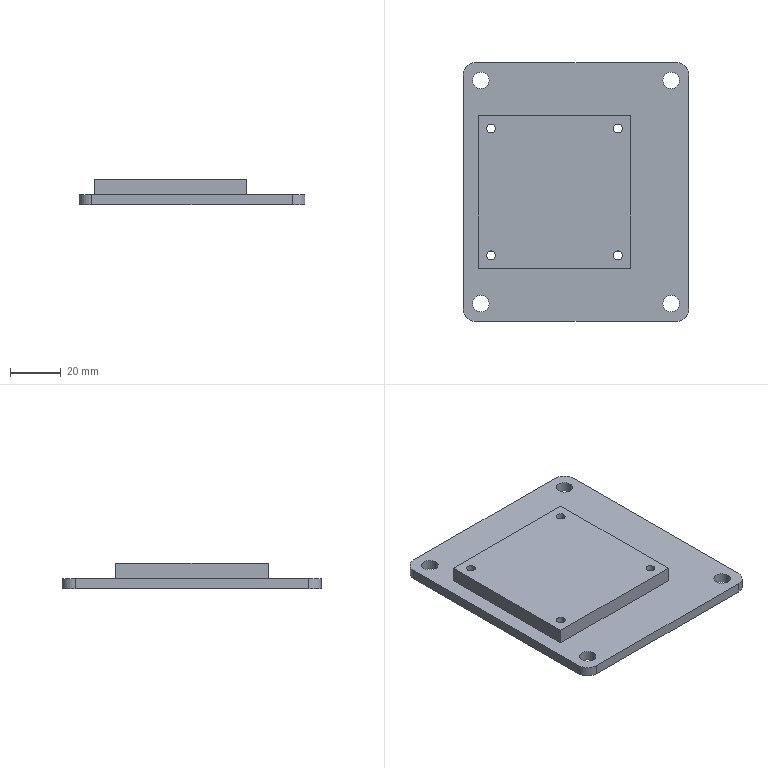CAM job | Mastercam | mm | 12 operations | part box 89 x 102 x 10
1. Facing | 24 - 100 平铣刀
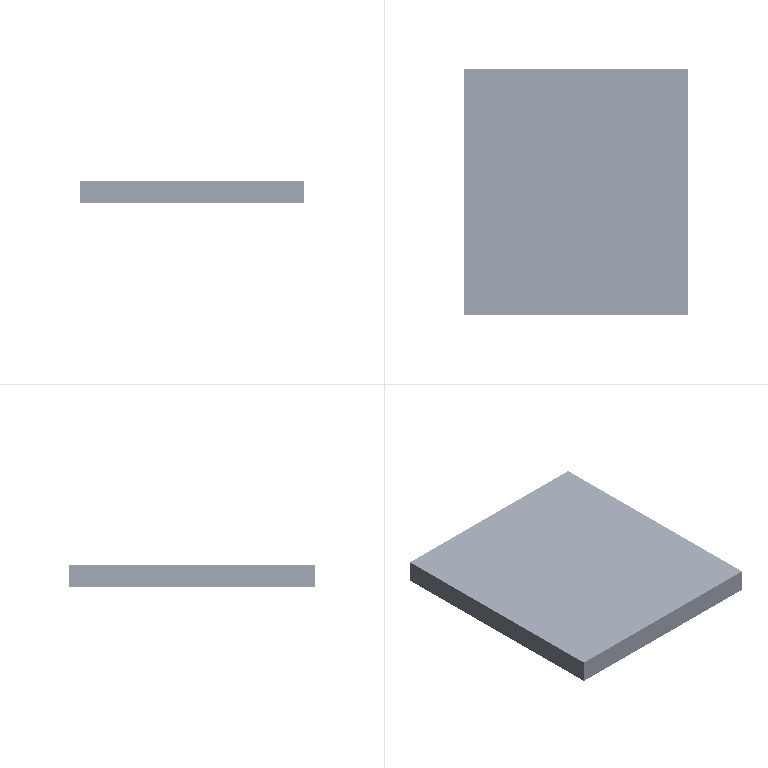2. 2D High Speed (2D Dynamic Mill) | 9 - 10 平铣刀
3. Contour (2D) | 10 - 10 平铣刀
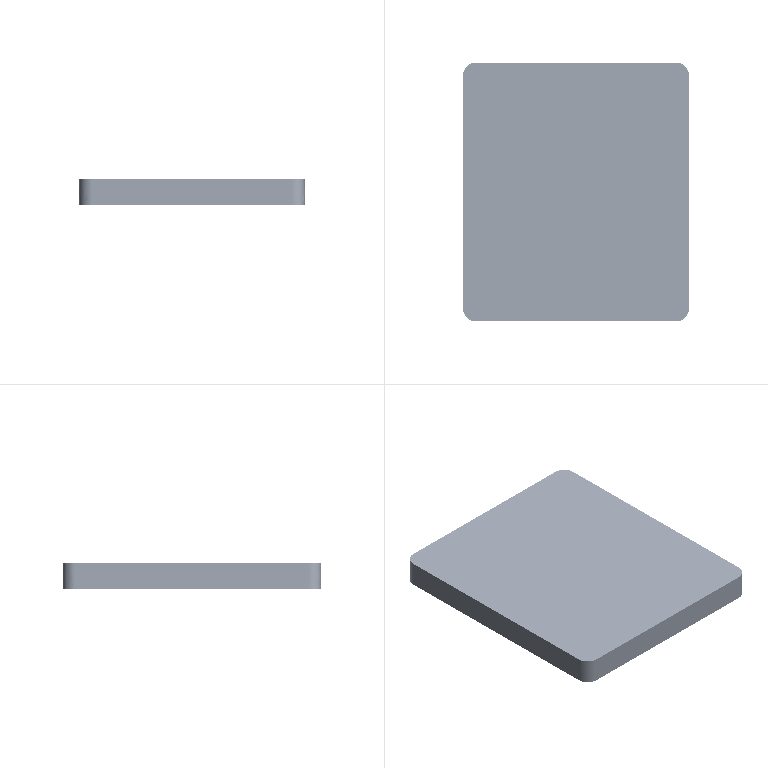4. Contour (2D chamfer) | 5 - 4 倒角刀
5. Facing | 9 - 10 平铣刀
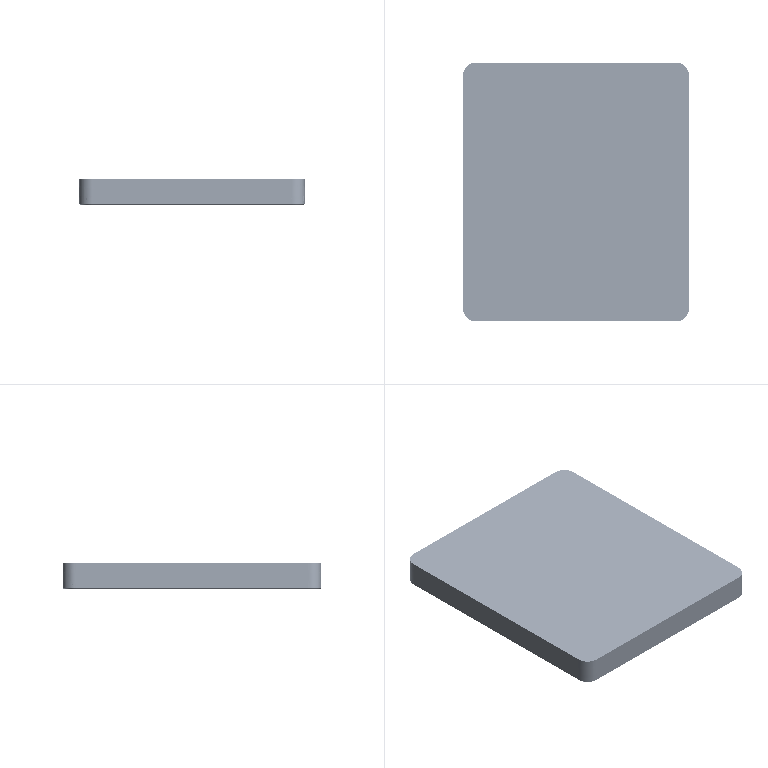6. 2D High Speed (2D Area Mill) | 9 - 10 平铣刀
7. 2D High Speed (2D Area Mill) | 10 - 10 平铣刀
8. Facing | 10 - 10 平铣刀
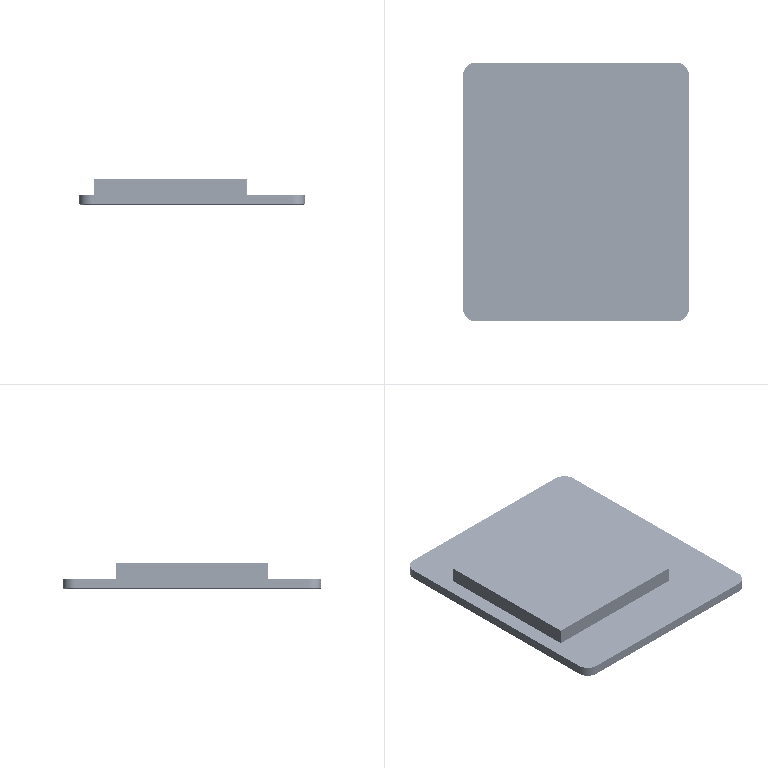9. Contour (2D) | 10 - 10 平铣刀
10. Drill/Counterbore | 5 - 4 倒角刀
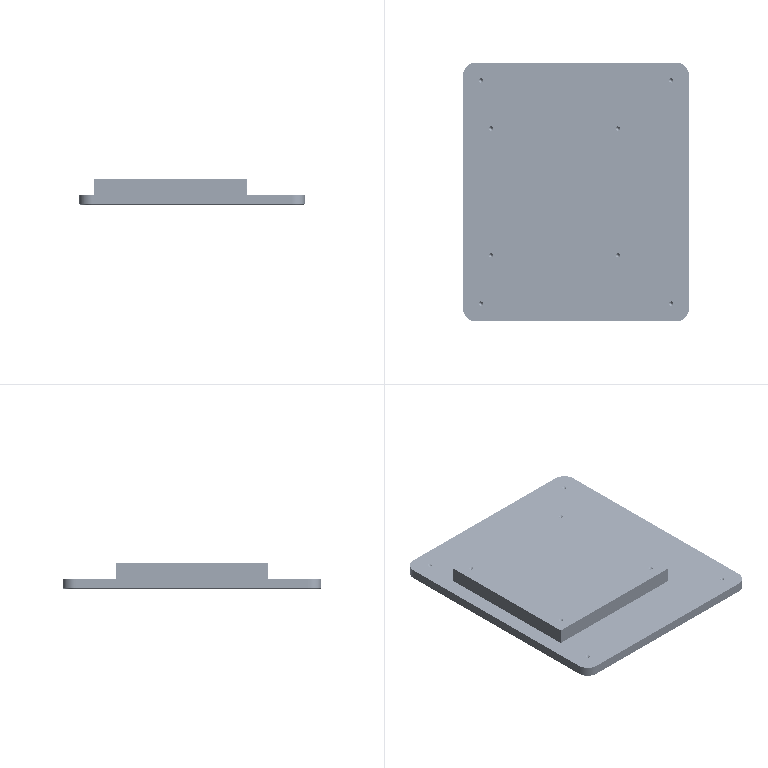11. Contour (2D chamfer) | 5 - 4 倒角刀
12. Contour (2D) | 10 - 10 平铣刀